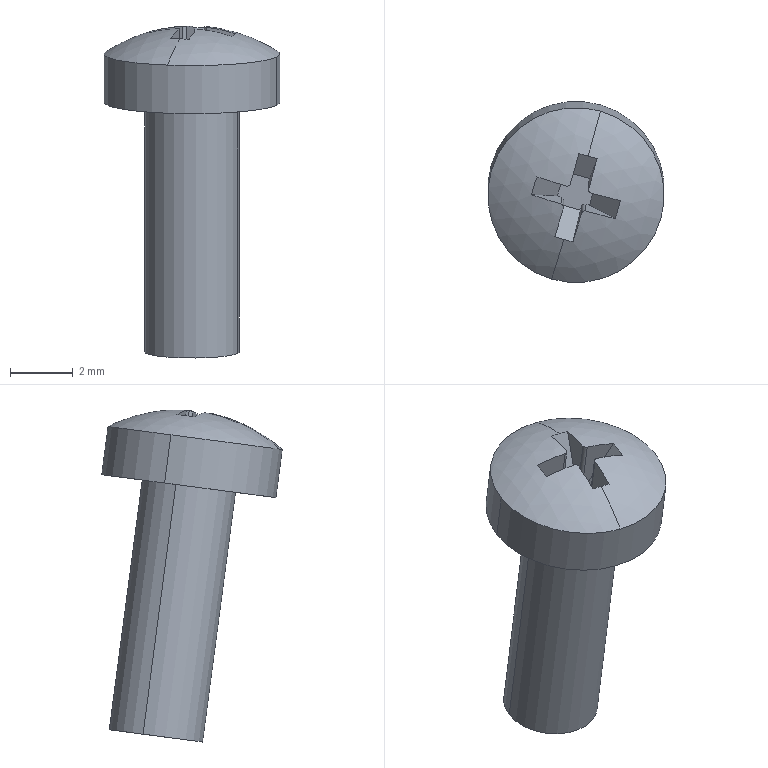Component | SolidWorks | SeedingAssemblyA-1_cross recessed pan head screws gb-12 | 1 solid | 25 faces | box 5.6 x 5.75 x 10.55 mm | volume 102 mm3 | plane 15 | cylinder 8 | sphere 2 | commonest cylinder face diameters 0.2 x4 5.6 x2 3 x2
STEP:
#1=COLOUR_RGB('',0.7922,0.8196,0.9333);
#2=FILL_AREA_STYLE_COLOUR('',#1);
#3=FILL_AREA_STYLE('',(#2));
#4=SURFACE_STYLE_FILL_AREA(#3);
#5=SURFACE_SIDE_STYLE('',(#4));
#6=SURFACE_STYLE_USAGE(.BOTH.,#5);
#7=PRESENTATION_STYLE_ASSIGNMENT((#6));
#8=CARTESIAN_POINT('',(3.542,-4.184,-2.825));
#9=VERTEX_POINT('',#8);
#10=CARTESIAN_POINT('',(3.466,-4.048,-2.807));
#11=VERTEX_POINT('',#10);
#12=CARTESIAN_POINT('',(3.572,-4.079,-2.811));
#13=DIRECTION('',(-0.,0.1306,-0.9914));
#14=DIRECTION('',(0.9609,-0.2744,-0.03615));
#15=AXIS2_PLACEMENT_3D('',#12,#13,#14);
#16=CIRCLE('',#15,0.1102);
#17=EDGE_CURVE('',#9,#11,#16,.T.);
#18=ORIENTED_EDGE('',*,*,#17,.T.);
#19=CARTESIAN_POINT('',(3.466,-4.04,-2.868));
#20=VERTEX_POINT('',#19);
#21=CARTESIAN_POINT('',(3.466,-4.029,-2.95));
#22=DIRECTION('',(-0.,0.1306,-0.9914));
#23=VECTOR('',#22,39.37);
#24=LINE('',#21,#23);
#25=EDGE_CURVE('',#11,#20,#24,.T.);
#26=ORIENTED_EDGE('',*,*,#25,.T.);
#27=CARTESIAN_POINT('',(3.678,-4.101,-2.876));
#28=VERTEX_POINT('',#27);
#29=CARTESIAN_POINT('',(3.572,-4.071,-2.872));
#30=DIRECTION('',(-0.,0.1306,-0.9914));
#31=DIRECTION('',(0.9609,-0.2744,-0.03615));
#32=AXIS2_PLACEMENT_3D('',#29,#30,#31);
#33=CIRCLE('',#32,0.1102);
#34=EDGE_CURVE('',#28,#20,#33,.T.);
#35=ORIENTED_EDGE('',*,*,#34,.F.);
#36=CARTESIAN_POINT('',(3.678,-4.109,-2.815));
#37=VERTEX_POINT('',#36);
#38=CARTESIAN_POINT('',(3.678,-4.09,-2.958));
#39=DIRECTION('',(-0.,0.1306,-0.9914));
#40=VECTOR('',#39,39.37);
#41=LINE('',#38,#40);
#42=EDGE_CURVE('',#37,#28,#41,.T.);
#43=ORIENTED_EDGE('',*,*,#42,.F.);
#44=CARTESIAN_POINT('',(3.572,-4.079,-2.811));
#45=DIRECTION('',(-0.,0.1306,-0.9914));
#46=DIRECTION('',(0.9609,-0.2744,-0.03615));
#47=AXIS2_PLACEMENT_3D('',#44,#45,#46);
#48=CIRCLE('',#47,0.1102);
#49=EDGE_CURVE('',#37,#9,#48,.T.);
#50=ORIENTED_EDGE('',*,*,#49,.T.);
#51=EDGE_LOOP('',(#18,#26,#35,#43,#50));
#52=FACE_OUTER_BOUND('',#51,.T.);
#53=CARTESIAN_POINT('',(3.572,-4.06,-2.954));
#54=DIRECTION('',(-0.,0.1306,-0.9914));
#55=DIRECTION('',(0.9609,-0.2744,-0.03615));
#56=AXIS2_PLACEMENT_3D('',#53,#54,#55);
#57=CYLINDRICAL_SURFACE('',#56,0.1102);
#58=ADVANCED_FACE('',(#52),#57,.T.);
#59=CARTESIAN_POINT('',(3.629,-4.087,-2.874));
#60=VERTEX_POINT('',#59);
#61=CARTESIAN_POINT('',(3.515,-4.054,-2.869));
#62=VERTEX_POINT('',#61);
#63=CARTESIAN_POINT('',(3.572,-4.071,-2.872));
#64=DIRECTION('',(-0.,0.1306,-0.9914));
#65=DIRECTION('',(0.9609,-0.2744,-0.03615));
#66=AXIS2_PLACEMENT_3D('',#63,#64,#65);
#67=CIRCLE('',#66,0.05906);
#68=EDGE_CURVE('',#60,#62,#67,.T.);
#69=ORIENTED_EDGE('',*,*,#68,.T.);
#70=CARTESIAN_POINT('',(3.515,-4.013,-3.182));
#71=VERTEX_POINT('',#70);
#72=CARTESIAN_POINT('',(3.515,-4.043,-2.952));
#73=DIRECTION('',(-0.,0.1306,-0.9914));
#74=VECTOR('',#73,39.37);
#75=LINE('',#72,#74);
#76=EDGE_CURVE('',#62,#71,#75,.T.);
#77=ORIENTED_EDGE('',*,*,#76,.T.);
#78=CARTESIAN_POINT('',(3.629,-4.046,-3.186));
#79=VERTEX_POINT('',#78);
#80=CARTESIAN_POINT('',(3.572,-4.029,-3.184));
#81=DIRECTION('',(-0.,0.1306,-0.9914));
#82=DIRECTION('',(0.9609,-0.2744,-0.03615));
#83=AXIS2_PLACEMENT_3D('',#80,#81,#82);
#84=CIRCLE('',#83,0.05906);
#85=EDGE_CURVE('',#79,#71,#84,.T.);
#86=ORIENTED_EDGE('',*,*,#85,.F.);
#87=CARTESIAN_POINT('',(3.629,-4.076,-2.956));
#88=DIRECTION('',(-0.,0.1306,-0.9914));
#89=VECTOR('',#88,39.37);
#90=LINE('',#87,#89);
#91=EDGE_CURVE('',#60,#79,#90,.T.);
#92=ORIENTED_EDGE('',*,*,#91,.F.);
#93=EDGE_LOOP('',(#69,#77,#86,#92));
#94=FACE_OUTER_BOUND('',#93,.T.);
#95=CARTESIAN_POINT('',(3.572,-4.06,-2.954));
#96=DIRECTION('',(-0.,0.1306,-0.9914));
#97=DIRECTION('',(0.9609,-0.2744,-0.03615));
#98=AXIS2_PLACEMENT_3D('',#95,#96,#97);
#99=CYLINDRICAL_SURFACE('',#98,0.05906);
#100=ADVANCED_FACE('',(#94),#99,.T.);
#101=CARTESIAN_POINT('',(3.576,-4.027,-2.779));
#102=VERTEX_POINT('',#101);
#103=CARTESIAN_POINT('',(3.587,-4.03,-2.779));
#104=VERTEX_POINT('',#103);
#105=CARTESIAN_POINT('',(3.561,-4.099,-2.955));
#106=DIRECTION('',(0.2397,0.8904,-0.387));
#107=DIRECTION('',(0.1384,0.3633,0.9214));
#108=AXIS2_PLACEMENT_3D('',#105,#106,#107);
#109=CIRCLE('',#108,0.1911);
#110=EDGE_CURVE('',#102,#104,#109,.T.);
#111=ORIENTED_EDGE('',*,*,#110,.T.);
#112=CARTESIAN_POINT('',(3.603,-3.973,-2.798));
#113=VERTEX_POINT('',#112);
#114=CARTESIAN_POINT('',(3.572,-4.057,-2.973));
#115=DIRECTION('',(-0.9609,0.2744,0.03615));
#116=DIRECTION('',(-0.2746,-0.9616,0.));
#117=AXIS2_PLACEMENT_3D('',#114,#115,#116);
#118=CIRCLE('',#117,0.1969);
#119=EDGE_CURVE('',#104,#113,#118,.T.);
#120=ORIENTED_EDGE('',*,*,#119,.T.);
#121=CARTESIAN_POINT('',(3.572,-4.079,-2.811));
#122=DIRECTION('',(-0.,0.1306,-0.9914));
#123=DIRECTION('',(0.9609,-0.2744,-0.03615));
#124=AXIS2_PLACEMENT_3D('',#121,#122,#123);
#125=CIRCLE('',#124,0.1102);
#126=EDGE_CURVE('',#11,#113,#125,.T.);
#127=ORIENTED_EDGE('',*,*,#126,.F.);
#128=ORIENTED_EDGE('',*,*,#17,.F.);
#129=CARTESIAN_POINT('',(3.557,-4.134,-2.792));
#130=VERTEX_POINT('',#129);
#131=CARTESIAN_POINT('',(3.572,-4.057,-2.973));
#132=DIRECTION('',(0.9609,-0.2744,-0.03615));
#133=DIRECTION('',(0.2746,0.9616,0.));
#134=AXIS2_PLACEMENT_3D('',#131,#132,#133);
#135=CIRCLE('',#134,0.1969);
#136=EDGE_CURVE('',#130,#9,#135,.T.);
#137=ORIENTED_EDGE('',*,*,#136,.F.);
#138=CARTESIAN_POINT('',(3.546,-4.13,-2.792));
#139=VERTEX_POINT('',#138);
#140=CARTESIAN_POINT('',(3.583,-4.021,-2.945));
#141=DIRECTION('',(-0.2397,-0.7598,-0.6044));
#142=DIRECTION('',(0.1384,0.5894,-0.7959));
#143=AXIS2_PLACEMENT_3D('',#140,#141,#142);
#144=CIRCLE('',#143,0.1911);
#145=EDGE_CURVE('',#130,#139,#144,.T.);
#146=ORIENTED_EDGE('',*,*,#145,.T.);
#147=CARTESIAN_POINT('',(3.556,-4.095,-2.78));
#148=VERTEX_POINT('',#147);
#149=CARTESIAN_POINT('',(3.561,-4.054,-2.973));
#150=DIRECTION('',(-0.9609,0.2744,0.03615));
#151=DIRECTION('',(-0.2768,-0.9527,-0.1255));
#152=AXIS2_PLACEMENT_3D('',#149,#150,#151);
#153=CIRCLE('',#152,0.1965);
#154=EDGE_CURVE('',#139,#148,#153,.T.);
#155=ORIENTED_EDGE('',*,*,#154,.T.);
#156=CARTESIAN_POINT('',(3.554,-4.09,-2.78));
#157=VERTEX_POINT('',#156);
#158=CARTESIAN_POINT('',(3.556,-4.095,-2.78));
#159=CARTESIAN_POINT('',(3.557,-4.094,-2.78));
#160=CARTESIAN_POINT('',(3.557,-4.094,-2.78));
#161=CARTESIAN_POINT('',(3.557,-4.093,-2.78));
#162=CARTESIAN_POINT('',(3.557,-4.093,-2.78));
#163=CARTESIAN_POINT('',(3.556,-4.092,-2.78));
#164=CARTESIAN_POINT('',(3.556,-4.092,-2.78));
#165=CARTESIAN_POINT('',(3.556,-4.092,-2.78));
#166=CARTESIAN_POINT('',(3.556,-4.091,-2.78));
#167=CARTESIAN_POINT('',(3.556,-4.091,-2.78));
#168=CARTESIAN_POINT('',(3.555,-4.091,-2.78));
#169=CARTESIAN_POINT('',(3.555,-4.09,-2.78));
#170=CARTESIAN_POINT('',(3.555,-4.09,-2.78));
#171=CARTESIAN_POINT('',(3.554,-4.09,-2.78));
#172=CARTESIAN_POINT('',(3.554,-4.09,-2.78));
#173=CARTESIAN_POINT('',(3.554,-4.09,-2.78));
#174=B_SPLINE_CURVE_WITH_KNOTS('',3,(#158,#159,#160,#161,#162,#163,#164,#165,#166,#167,#168,#169,#170,#171,#172,#173),.UNSPECIFIED.,.F.,.F.,(4,3,3,3,3,4),(0.,0.00003353,0.00006707,0.0001005,0.0001339,0.0001564),.UNSPECIFIED.);
#175=EDGE_CURVE('',#148,#157,#174,.T.);
#176=ORIENTED_EDGE('',*,*,#175,.T.);
#177=CARTESIAN_POINT('',(3.517,-4.078,-2.785));
#178=VERTEX_POINT('',#177);
#179=CARTESIAN_POINT('',(3.569,-4.068,-2.975));
#180=DIRECTION('',(-0.2768,-0.9527,-0.1255));
#181=DIRECTION('',(0.9609,-0.2744,-0.03615));
#182=AXIS2_PLACEMENT_3D('',#179,#180,#181);
#183=CIRCLE('',#182,0.1965);
#184=EDGE_CURVE('',#157,#178,#183,.T.);
#185=ORIENTED_EDGE('',*,*,#184,.T.);
#186=CARTESIAN_POINT('',(3.523,-4.056,-2.782));
#187=VERTEX_POINT('',#186);
#188=CARTESIAN_POINT('',(3.611,-4.072,-2.951));
#189=DIRECTION('',(-0.8322,0.303,-0.4644));
#190=DIRECTION('',(-0.4805,0.02413,0.8767));
#191=AXIS2_PLACEMENT_3D('',#188,#189,#190);
#192=CIRCLE('',#191,0.1911);
#193=EDGE_CURVE('',#178,#187,#192,.T.);
#194=ORIENTED_EDGE('',*,*,#193,.T.);
#195=CARTESIAN_POINT('',(3.56,-4.067,-2.777));
#196=VERTEX_POINT('',#195);
#197=CARTESIAN_POINT('',(3.575,-4.046,-2.972));
#198=DIRECTION('',(0.2768,0.9527,0.1255));
#199=DIRECTION('',(-0.9609,0.2744,0.03615));
#200=AXIS2_PLACEMENT_3D('',#197,#198,#199);
#201=CIRCLE('',#200,0.1965);
#202=EDGE_CURVE('',#187,#196,#201,.T.);
#203=ORIENTED_EDGE('',*,*,#202,.T.);
#204=CARTESIAN_POINT('',(3.565,-4.065,-2.777));
#205=VERTEX_POINT('',#204);
#206=CARTESIAN_POINT('',(3.56,-4.067,-2.777));
#207=CARTESIAN_POINT('',(3.561,-4.067,-2.777));
#208=CARTESIAN_POINT('',(3.561,-4.067,-2.777));
#209=CARTESIAN_POINT('',(3.562,-4.067,-2.777));
#210=CARTESIAN_POINT('',(3.562,-4.067,-2.777));
#211=CARTESIAN_POINT('',(3.562,-4.067,-2.777));
#212=CARTESIAN_POINT('',(3.563,-4.067,-2.777));
#213=CARTESIAN_POINT('',(3.563,-4.067,-2.777));
#214=CARTESIAN_POINT('',(3.564,-4.067,-2.777));
#215=CARTESIAN_POINT('',(3.564,-4.066,-2.777));
#216=CARTESIAN_POINT('',(3.564,-4.066,-2.777));
#217=CARTESIAN_POINT('',(3.565,-4.066,-2.777));
#218=CARTESIAN_POINT('',(3.565,-4.065,-2.777));
#219=CARTESIAN_POINT('',(3.565,-4.065,-2.777));
#220=CARTESIAN_POINT('',(3.565,-4.065,-2.777));
#221=CARTESIAN_POINT('',(3.565,-4.065,-2.777));
#222=B_SPLINE_CURVE_WITH_KNOTS('',3,(#206,#207,#208,#209,#210,#211,#212,#213,#214,#215,#216,#217,#218,#219,#220,#221),.UNSPECIFIED.,.F.,.F.,(4,3,3,3,3,4),(0.,0.00003353,0.00006707,0.0001005,0.0001339,0.0001564),.UNSPECIFIED.);
#223=EDGE_CURVE('',#196,#205,#222,.T.);
#224=ORIENTED_EDGE('',*,*,#223,.T.);
#225=CARTESIAN_POINT('',(3.561,-4.054,-2.973));
#226=DIRECTION('',(-0.9609,0.2744,0.03615));
#227=DIRECTION('',(-0.2768,-0.9527,-0.1255));
#228=AXIS2_PLACEMENT_3D('',#225,#226,#227);
#229=CIRCLE('',#228,0.1965);
#230=EDGE_CURVE('',#205,#102,#229,.T.);
#231=ORIENTED_EDGE('',*,*,#230,.T.);
#232=EDGE_LOOP('',(#111,#120,#127,#128,#137,#146,#155,#176,#185,#194,#203,#224,#231));
#233=FACE_OUTER_BOUND('',#232,.T.);
#234=CARTESIAN_POINT('',(3.572,-4.057,-2.973));
#235=DIRECTION('',(-0.9609,0.2744,0.03615));
#236=DIRECTION('',(-0.2768,-0.9527,-0.1255));
#237=AXIS2_PLACEMENT_3D('',#234,#235,#236);
#238=SPHERICAL_SURFACE('',#237,0.1969);
#239=ADVANCED_FACE('',(#233),#238,.T.);
#240=ORIENTED_EDGE('',*,*,#119,.F.);
#241=CARTESIAN_POINT('',(3.599,-4.033,-2.779));
#242=VERTEX_POINT('',#241);
#243=CARTESIAN_POINT('',(3.561,-4.099,-2.955));
#244=DIRECTION('',(0.2397,0.8904,-0.387));
#245=DIRECTION('',(0.1384,0.3633,0.9214));
#246=AXIS2_PLACEMENT_3D('',#243,#244,#245);
#247=CIRCLE('',#246,0.1911);
#248=EDGE_CURVE('',#104,#242,#247,.T.);
#249=ORIENTED_EDGE('',*,*,#248,.T.);
#250=CARTESIAN_POINT('',(3.588,-4.071,-2.777));
#251=VERTEX_POINT('',#250);
#252=CARTESIAN_POINT('',(3.583,-4.06,-2.974));
#253=DIRECTION('',(0.9609,-0.2744,-0.03615));
#254=DIRECTION('',(0.,0.1306,-0.9914));
#255=AXIS2_PLACEMENT_3D('',#252,#253,#254);
#256=CIRCLE('',#255,0.1965);
#257=EDGE_CURVE('',#242,#251,#256,.T.);
#258=ORIENTED_EDGE('',*,*,#257,.T.);
#259=CARTESIAN_POINT('',(3.591,-4.076,-2.778));
#260=VERTEX_POINT('',#259);
#261=CARTESIAN_POINT('',(3.588,-4.071,-2.777));
#262=CARTESIAN_POINT('',(3.588,-4.071,-2.777));
#263=CARTESIAN_POINT('',(3.588,-4.072,-2.777));
#264=CARTESIAN_POINT('',(3.588,-4.072,-2.777));
#265=CARTESIAN_POINT('',(3.588,-4.073,-2.777));
#266=CARTESIAN_POINT('',(3.588,-4.073,-2.778));
#267=CARTESIAN_POINT('',(3.588,-4.074,-2.778));
#268=CARTESIAN_POINT('',(3.588,-4.074,-2.778));
#269=CARTESIAN_POINT('',(3.588,-4.074,-2.778));
#270=CARTESIAN_POINT('',(3.589,-4.075,-2.778));
#271=CARTESIAN_POINT('',(3.589,-4.075,-2.778));
#272=CARTESIAN_POINT('',(3.589,-4.075,-2.778));
#273=CARTESIAN_POINT('',(3.59,-4.076,-2.778));
#274=CARTESIAN_POINT('',(3.59,-4.076,-2.778));
#275=CARTESIAN_POINT('',(3.59,-4.076,-2.778));
#276=CARTESIAN_POINT('',(3.591,-4.076,-2.778));
#277=B_SPLINE_CURVE_WITH_KNOTS('',3,(#261,#262,#263,#264,#265,#266,#267,#268,#269,#270,#271,#272,#273,#274,#275,#276),.UNSPECIFIED.,.F.,.F.,(4,3,3,3,3,4),(0.,0.00003353,0.00006707,0.0001005,0.0001339,0.0001564),.UNSPECIFIED.);
#278=EDGE_CURVE('',#251,#260,#277,.T.);
#279=ORIENTED_EDGE('',*,*,#278,.T.);
#280=CARTESIAN_POINT('',(3.628,-4.086,-2.786));
#281=VERTEX_POINT('',#280);
#282=CARTESIAN_POINT('',(3.575,-4.046,-2.972));
#283=DIRECTION('',(0.2768,0.9527,0.1255));
#284=DIRECTION('',(-0.9609,0.2744,0.03615));
#285=AXIS2_PLACEMENT_3D('',#282,#283,#284);
#286=CIRCLE('',#285,0.1965);
#287=EDGE_CURVE('',#260,#281,#286,.T.);
#288=ORIENTED_EDGE('',*,*,#287,.T.);
#289=CARTESIAN_POINT('',(3.621,-4.108,-2.789));
#290=VERTEX_POINT('',#289);
#291=CARTESIAN_POINT('',(3.533,-4.049,-2.948));
#292=DIRECTION('',(0.8322,-0.1724,-0.527));
#293=DIRECTION('',(-0.4805,0.2503,-0.8405));
#294=AXIS2_PLACEMENT_3D('',#291,#292,#293);
#295=CIRCLE('',#294,0.1911);
#296=EDGE_CURVE('',#281,#290,#295,.T.);
#297=ORIENTED_EDGE('',*,*,#296,.T.);
#298=CARTESIAN_POINT('',(3.584,-4.098,-2.781));
#299=VERTEX_POINT('',#298);
#300=CARTESIAN_POINT('',(3.569,-4.068,-2.975));
#301=DIRECTION('',(-0.2768,-0.9527,-0.1255));
#302=DIRECTION('',(0.9609,-0.2744,-0.03615));
#303=AXIS2_PLACEMENT_3D('',#300,#301,#302);
#304=CIRCLE('',#303,0.1965);
#305=EDGE_CURVE('',#290,#299,#304,.T.);
#306=ORIENTED_EDGE('',*,*,#305,.T.);
#307=CARTESIAN_POINT('',(3.579,-4.101,-2.781));
#308=VERTEX_POINT('',#307);
#309=CARTESIAN_POINT('',(3.584,-4.098,-2.781));
#310=CARTESIAN_POINT('',(3.584,-4.098,-2.781));
#311=CARTESIAN_POINT('',(3.583,-4.098,-2.781));
#312=CARTESIAN_POINT('',(3.583,-4.098,-2.781));
#313=CARTESIAN_POINT('',(3.582,-4.098,-2.781));
#314=CARTESIAN_POINT('',(3.582,-4.098,-2.781));
#315=CARTESIAN_POINT('',(3.581,-4.099,-2.781));
#316=CARTESIAN_POINT('',(3.581,-4.099,-2.781));
#317=CARTESIAN_POINT('',(3.581,-4.099,-2.781));
#318=CARTESIAN_POINT('',(3.58,-4.099,-2.781));
#319=CARTESIAN_POINT('',(3.58,-4.1,-2.781));
#320=CARTESIAN_POINT('',(3.58,-4.1,-2.781));
#321=CARTESIAN_POINT('',(3.579,-4.1,-2.781));
#322=CARTESIAN_POINT('',(3.579,-4.1,-2.781));
#323=CARTESIAN_POINT('',(3.579,-4.101,-2.781));
#324=CARTESIAN_POINT('',(3.579,-4.101,-2.781));
#325=B_SPLINE_CURVE_WITH_KNOTS('',3,(#309,#310,#311,#312,#313,#314,#315,#316,#317,#318,#319,#320,#321,#322,#323,#324),.UNSPECIFIED.,.F.,.F.,(4,3,3,3,3,4),(0.,0.00003353,0.00006707,0.0001005,0.0001339,0.0001564),.UNSPECIFIED.);
#326=EDGE_CURVE('',#299,#308,#325,.T.);
#327=ORIENTED_EDGE('',*,*,#326,.T.);
#328=CARTESIAN_POINT('',(3.568,-4.137,-2.793));
#329=VERTEX_POINT('',#328);
#330=CARTESIAN_POINT('',(3.583,-4.06,-2.974));
#331=DIRECTION('',(0.9609,-0.2744,-0.03615));
#332=DIRECTION('',(0.,0.1306,-0.9914));
#333=AXIS2_PLACEMENT_3D('',#330,#331,#332);
#334=CIRCLE('',#333,0.1965);
#335=EDGE_CURVE('',#308,#329,#334,.T.);
#336=ORIENTED_EDGE('',*,*,#335,.T.);
#337=CARTESIAN_POINT('',(3.583,-4.021,-2.945));
#338=DIRECTION('',(-0.2397,-0.7598,-0.6044));
#339=DIRECTION('',(0.1384,0.5894,-0.7959));
#340=AXIS2_PLACEMENT_3D('',#337,#338,#339);
#341=CIRCLE('',#340,0.1911);
#342=EDGE_CURVE('',#329,#130,#341,.T.);
#343=ORIENTED_EDGE('',*,*,#342,.T.);
#344=ORIENTED_EDGE('',*,*,#136,.T.);
#345=ORIENTED_EDGE('',*,*,#49,.F.);
#346=CARTESIAN_POINT('',(3.572,-4.079,-2.811));
#347=DIRECTION('',(-0.,0.1306,-0.9914));
#348=DIRECTION('',(0.9609,-0.2744,-0.03615));
#349=AXIS2_PLACEMENT_3D('',#346,#347,#348);
#350=CIRCLE('',#349,0.1102);
#351=EDGE_CURVE('',#113,#37,#350,.T.);
#352=ORIENTED_EDGE('',*,*,#351,.F.);
#353=EDGE_LOOP('',(#240,#249,#258,#279,#288,#297,#306,#327,#336,#343,#344,#345,#352));
#354=FACE_OUTER_BOUND('',#353,.T.);
#355=CARTESIAN_POINT('',(3.572,-4.057,-2.973));
#356=DIRECTION('',(-0.9609,0.2744,0.03615));
#357=DIRECTION('',(-0.2768,-0.9527,-0.1255));
#358=AXIS2_PLACEMENT_3D('',#355,#356,#357);
#359=SPHERICAL_SURFACE('',#358,0.1969);
#360=ADVANCED_FACE('',(#354),#359,.T.);
#361=ORIENTED_EDGE('',*,*,#85,.T.);
#362=CARTESIAN_POINT('',(3.572,-4.029,-3.184));
#363=DIRECTION('',(-0.,0.1306,-0.9914));
#364=DIRECTION('',(0.9609,-0.2744,-0.03615));
#365=AXIS2_PLACEMENT_3D('',#362,#363,#364);
#366=CIRCLE('',#365,0.05906);
#367=EDGE_CURVE('',#71,#79,#366,.T.);
#368=ORIENTED_EDGE('',*,*,#367,.T.);
#369=EDGE_LOOP('',(#361,#368));
#370=FACE_OUTER_BOUND('',#369,.T.);
#371=CARTESIAN_POINT('',(3.556,-4.086,-3.191));
#372=DIRECTION('',(-0.,0.1306,-0.9914));
#373=DIRECTION('',(0.9609,-0.2744,-0.03615));
#374=AXIS2_PLACEMENT_3D('',#371,#372,#373);
#375=PLANE('',#374);
#376=ADVANCED_FACE('',(#370),#375,.T.);
#377=ORIENTED_EDGE('',*,*,#76,.F.);
#378=CARTESIAN_POINT('',(3.572,-4.071,-2.872));
#379=DIRECTION('',(-0.,0.1306,-0.9914));
#380=DIRECTION('',(0.9609,-0.2744,-0.03615));
#381=AXIS2_PLACEMENT_3D('',#378,#379,#380);
#382=CIRCLE('',#381,0.05906);
#383=EDGE_CURVE('',#62,#60,#382,.T.);
#384=ORIENTED_EDGE('',*,*,#383,.T.);
#385=ORIENTED_EDGE('',*,*,#91,.T.);
#386=ORIENTED_EDGE('',*,*,#367,.F.);
#387=EDGE_LOOP('',(#377,#384,#385,#386));
#388=FACE_OUTER_BOUND('',#387,.T.);
#389=CARTESIAN_POINT('',(3.572,-4.06,-2.954));
#390=DIRECTION('',(-0.,0.1306,-0.9914));
#391=DIRECTION('',(0.9609,-0.2744,-0.03615));
#392=AXIS2_PLACEMENT_3D('',#389,#390,#391);
#393=CYLINDRICAL_SURFACE('',#392,0.05906);
#394=ADVANCED_FACE('',(#388),#393,.T.);
#395=ORIENTED_EDGE('',*,*,#34,.T.);
#396=CARTESIAN_POINT('',(3.572,-4.071,-2.872));
#397=DIRECTION('',(-0.,0.1306,-0.9914));
#398=DIRECTION('',(0.9609,-0.2744,-0.03615));
#399=AXIS2_PLACEMENT_3D('',#396,#397,#398);
#400=CIRCLE('',#399,0.1102);
#401=EDGE_CURVE('',#20,#28,#400,.T.);
#402=ORIENTED_EDGE('',*,*,#401,.T.);
#403=EDGE_LOOP('',(#395,#402));
#404=FACE_OUTER_BOUND('',#403,.T.);
#405=ORIENTED_EDGE('',*,*,#68,.F.);
#406=ORIENTED_EDGE('',*,*,#383,.F.);
#407=EDGE_LOOP('',(#405,#406));
#408=FACE_BOUND('',#407,.T.);
#409=CARTESIAN_POINT('',(3.552,-4.138,-2.88));
#410=DIRECTION('',(-0.,0.1306,-0.9914));
#411=DIRECTION('',(0.9609,-0.2744,-0.03615));
#412=AXIS2_PLACEMENT_3D('',#409,#410,#411);
#413=PLANE('',#412);
#414=ADVANCED_FACE('',(#404,#408),#413,.T.);
#415=ORIENTED_EDGE('',*,*,#25,.F.);
#416=ORIENTED_EDGE('',*,*,#126,.T.);
#417=ORIENTED_EDGE('',*,*,#351,.T.);
#418=ORIENTED_EDGE('',*,*,#42,.T.);
#419=ORIENTED_EDGE('',*,*,#401,.F.);
#420=EDGE_LOOP('',(#415,#416,#417,#418,#419));
#421=FACE_OUTER_BOUND('',#420,.T.);
#422=CARTESIAN_POINT('',(3.572,-4.06,-2.954));
#423=DIRECTION('',(-0.,0.1306,-0.9914));
#424=DIRECTION('',(0.9609,-0.2744,-0.03615));
#425=AXIS2_PLACEMENT_3D('',#422,#423,#424);
#426=CYLINDRICAL_SURFACE('',#425,0.1102);
#427=ADVANCED_FACE('',(#421),#426,.T.);
#428=ORIENTED_EDGE('',*,*,#184,.F.);
#429=CARTESIAN_POINT('',(3.554,-4.081,-2.844));
#430=VERTEX_POINT('',#429);
#431=CARTESIAN_POINT('',(3.554,-4.081,-2.844));
#432=DIRECTION('',(-0.,0.1306,-0.9914));
#433=VECTOR('',#432,39.37);
#434=LINE('',#431,#433);
#435=EDGE_CURVE('',#157,#430,#434,.T.);
#436=ORIENTED_EDGE('',*,*,#435,.T.);
#437=CARTESIAN_POINT('',(3.549,-4.08,-2.844));
#438=VERTEX_POINT('',#437);
#439=CARTESIAN_POINT('',(3.557,-4.082,-2.845));
#440=DIRECTION('',(-0.9609,0.2744,0.03615));
#441=VECTOR('',#440,39.37);
#442=LINE('',#439,#441);
#443=EDGE_CURVE('',#430,#438,#442,.T.);
#444=ORIENTED_EDGE('',*,*,#443,.T.);
#445=CARTESIAN_POINT('',(3.512,-4.078,-2.777));
#446=DIRECTION('',(-0.4805,0.02413,0.8767));
#447=VECTOR('',#446,39.37);
#448=LINE('',#445,#447);
#449=EDGE_CURVE('',#438,#178,#448,.T.);
#450=ORIENTED_EDGE('',*,*,#449,.T.);
#451=EDGE_LOOP('',(#428,#436,#444,#450));
#452=FACE_OUTER_BOUND('',#451,.T.);
#453=CARTESIAN_POINT('',(3.557,-4.082,-2.845));
#454=DIRECTION('',(0.2768,0.9527,0.1255));
#455=DIRECTION('',(0.9609,-0.2744,-0.03615));
#456=AXIS2_PLACEMENT_3D('',#453,#454,#455);
#457=PLANE('',#456);
#458=ADVANCED_FACE('',(#452),#457,.T.);
#459=ORIENTED_EDGE('',*,*,#449,.F.);
#460=CARTESIAN_POINT('',(3.555,-4.057,-2.841));
#461=VERTEX_POINT('',#460);
#462=CARTESIAN_POINT('',(3.549,-4.08,-2.844));
#463=DIRECTION('',(0.2768,0.9527,0.1255));
#464=VECTOR('',#463,39.37);
#465=LINE('',#462,#464);
#466=EDGE_CURVE('',#438,#461,#465,.T.);
#467=ORIENTED_EDGE('',*,*,#466,.T.);
#468=CARTESIAN_POINT('',(3.557,-4.057,-2.845));
#469=DIRECTION('',(-0.4805,0.02413,0.8767));
#470=VECTOR('',#469,39.37);
#471=LINE('',#468,#470);
#472=EDGE_CURVE('',#461,#187,#471,.T.);
#473=ORIENTED_EDGE('',*,*,#472,.T.);
#474=ORIENTED_EDGE('',*,*,#193,.F.);
#475=EDGE_LOOP('',(#459,#467,#473,#474));
#476=FACE_OUTER_BOUND('',#475,.T.);
#477=CARTESIAN_POINT('',(3.515,-4.067,-2.776));
#478=DIRECTION('',(0.8322,-0.303,0.4644));
#479=DIRECTION('',(-0.4805,0.02413,0.8767));
#480=AXIS2_PLACEMENT_3D('',#477,#478,#479);
#481=PLANE('',#480);
#482=ADVANCED_FACE('',(#476),#481,.T.);
#483=CARTESIAN_POINT('',(3.56,-4.059,-2.841));
#484=VERTEX_POINT('',#483);
#485=CARTESIAN_POINT('',(3.564,-4.06,-2.842));
#486=DIRECTION('',(0.9609,-0.2744,-0.03615));
#487=VECTOR('',#486,39.37);
#488=LINE('',#485,#487);
#489=EDGE_CURVE('',#461,#484,#488,.T.);
#490=ORIENTED_EDGE('',*,*,#489,.T.);
#491=CARTESIAN_POINT('',(3.56,-4.059,-2.841));
#492=DIRECTION('',(0.,-0.1306,0.9914));
#493=VECTOR('',#492,39.37);
#494=LINE('',#491,#493);
#495=EDGE_CURVE('',#484,#196,#494,.T.);
#496=ORIENTED_EDGE('',*,*,#495,.T.);
#497=ORIENTED_EDGE('',*,*,#202,.F.);
#498=ORIENTED_EDGE('',*,*,#472,.F.);
#499=EDGE_LOOP('',(#490,#496,#497,#498));
#500=FACE_OUTER_BOUND('',#499,.T.);
#501=CARTESIAN_POINT('',(3.564,-4.06,-2.842));
#502=DIRECTION('',(-0.2768,-0.9527,-0.1255));
#503=DIRECTION('',(-0.9609,0.2744,0.03615));
#504=AXIS2_PLACEMENT_3D('',#501,#502,#503);
#505=PLANE('',#504);
#506=ADVANCED_FACE('',(#500),#505,.T.);
#507=ORIENTED_EDGE('',*,*,#230,.F.);
#508=CARTESIAN_POINT('',(3.565,-4.056,-2.841));
#509=VERTEX_POINT('',#508);
#510=CARTESIAN_POINT('',(3.565,-4.056,-2.841));
#511=DIRECTION('',(-0.,0.1306,-0.9914));
#512=VECTOR('',#511,39.37);
#513=LINE('',#510,#512);
#514=EDGE_CURVE('',#205,#509,#513,.T.);
#515=ORIENTED_EDGE('',*,*,#514,.T.);
#516=CARTESIAN_POINT('',(3.567,-4.051,-2.84));
#517=VERTEX_POINT('',#516);
#518=CARTESIAN_POINT('',(3.564,-4.06,-2.842));
#519=DIRECTION('',(0.2768,0.9527,0.1255));
#520=VECTOR('',#519,39.37);
#521=LINE('',#518,#520);
#522=EDGE_CURVE('',#509,#517,#521,.T.);
#523=ORIENTED_EDGE('',*,*,#522,.T.);
#524=CARTESIAN_POINT('',(3.577,-4.023,-2.77));
#525=DIRECTION('',(0.1384,0.3633,0.9214));
#526=VECTOR('',#525,39.37);
#527=LINE('',#524,#526);
#528=EDGE_CURVE('',#517,#102,#527,.T.);
#529=ORIENTED_EDGE('',*,*,#528,.T.);
#530=EDGE_LOOP('',(#507,#515,#523,#529));
#531=FACE_OUTER_BOUND('',#530,.T.);
#532=CARTESIAN_POINT('',(3.564,-4.06,-2.842));
#533=DIRECTION('',(0.9609,-0.2744,-0.03615));
#534=DIRECTION('',(-0.2768,-0.9527,-0.1255));
#535=AXIS2_PLACEMENT_3D('',#532,#533,#534);
#536=PLANE('',#535);
#537=ADVANCED_FACE('',(#531),#536,.T.);
#538=ORIENTED_EDGE('',*,*,#528,.F.);
#539=CARTESIAN_POINT('',(3.589,-4.058,-2.841));
#540=VERTEX_POINT('',#539);
#541=CARTESIAN_POINT('',(3.567,-4.051,-2.84));
#542=DIRECTION('',(0.9609,-0.2744,-0.03615));
#543=VECTOR('',#542,39.37);
#544=LINE('',#541,#543);
#545=EDGE_CURVE('',#517,#540,#544,.T.);
#546=ORIENTED_EDGE('',*,*,#545,.T.);
#547=CARTESIAN_POINT('',(3.589,-4.059,-2.845));
#548=DIRECTION('',(0.1384,0.3633,0.9214));
#549=VECTOR('',#548,39.37);
#550=LINE('',#547,#549);
#551=EDGE_CURVE('',#540,#242,#550,.T.);
#552=ORIENTED_EDGE('',*,*,#551,.T.);
#553=ORIENTED_EDGE('',*,*,#248,.F.);
#554=ORIENTED_EDGE('',*,*,#110,.F.);
#555=EDGE_LOOP('',(#538,#546,#552,#553,#554));
#556=FACE_OUTER_BOUND('',#555,.T.);
#557=CARTESIAN_POINT('',(3.588,-4.027,-2.771));
#558=DIRECTION('',(-0.2397,-0.8904,0.387));
#559=DIRECTION('',(0.1384,0.3633,0.9214));
#560=AXIS2_PLACEMENT_3D('',#557,#558,#559);
#561=PLANE('',#560);
#562=ADVANCED_FACE('',(#556),#561,.T.);
#563=CARTESIAN_POINT('',(3.588,-4.063,-2.842));
#564=VERTEX_POINT('',#563);
#565=CARTESIAN_POINT('',(3.587,-4.066,-2.842));
#566=DIRECTION('',(-0.2768,-0.9527,-0.1255));
#567=VECTOR('',#566,39.37);
#568=LINE('',#565,#567);
#569=EDGE_CURVE('',#540,#564,#568,.T.);
#570=ORIENTED_EDGE('',*,*,#569,.T.);
#571=CARTESIAN_POINT('',(3.588,-4.063,-2.842));
#572=DIRECTION('',(0.,-0.1306,0.9914));
#573=VECTOR('',#572,39.37);
#574=LINE('',#571,#573);
#575=EDGE_CURVE('',#564,#251,#574,.T.);
#576=ORIENTED_EDGE('',*,*,#575,.T.);
#577=ORIENTED_EDGE('',*,*,#257,.F.);
#578=ORIENTED_EDGE('',*,*,#551,.F.);
#579=EDGE_LOOP('',(#570,#576,#577,#578));
#580=FACE_OUTER_BOUND('',#579,.T.);
#581=CARTESIAN_POINT('',(3.587,-4.066,-2.842));
#582=DIRECTION('',(-0.9609,0.2744,0.03615));
#583=DIRECTION('',(-0.,0.1306,-0.9914));
#584=AXIS2_PLACEMENT_3D('',#581,#582,#583);
#585=PLANE('',#584);
#586=ADVANCED_FACE('',(#580),#585,.T.);
#587=ORIENTED_EDGE('',*,*,#287,.F.);
#588=CARTESIAN_POINT('',(3.591,-4.067,-2.843));
#589=VERTEX_POINT('',#588);
#590=CARTESIAN_POINT('',(3.591,-4.067,-2.843));
#591=DIRECTION('',(-0.,0.1306,-0.9914));
#592=VECTOR('',#591,39.37);
#593=LINE('',#590,#592);
#594=EDGE_CURVE('',#260,#589,#593,.T.);
#595=ORIENTED_EDGE('',*,*,#594,.T.);
#596=CARTESIAN_POINT('',(3.595,-4.069,-2.843));
#597=VERTEX_POINT('',#596);
#598=CARTESIAN_POINT('',(3.587,-4.066,-2.842));
#599=DIRECTION('',(0.9609,-0.2744,-0.03615));
#600=VECTOR('',#599,39.37);
#601=LINE('',#598,#600);
#602=EDGE_CURVE('',#589,#597,#601,.T.);
#603=ORIENTED_EDGE('',*,*,#602,.T.);
#604=CARTESIAN_POINT('',(3.632,-4.088,-2.779));
#605=DIRECTION('',(0.4805,-0.2503,0.8405));
#606=VECTOR('',#605,39.37);
#607=LINE('',#604,#606);
#608=EDGE_CURVE('',#597,#281,#607,.T.);
#609=ORIENTED_EDGE('',*,*,#608,.T.);
#610=EDGE_LOOP('',(#587,#595,#603,#609));
#611=FACE_OUTER_BOUND('',#610,.T.);
#612=CARTESIAN_POINT('',(3.587,-4.066,-2.842));
#613=DIRECTION('',(-0.2768,-0.9527,-0.1255));
#614=DIRECTION('',(-0.9609,0.2744,0.03615));
#615=AXIS2_PLACEMENT_3D('',#612,#613,#614);
#616=PLANE('',#615);
#617=ADVANCED_FACE('',(#611),#616,.T.);
#618=ORIENTED_EDGE('',*,*,#608,.F.);
#619=CARTESIAN_POINT('',(3.589,-4.091,-2.846));
#620=VERTEX_POINT('',#619);
#621=CARTESIAN_POINT('',(3.589,-4.091,-2.846));
#622=DIRECTION('',(-0.2768,-0.9527,-0.1255));
#623=VECTOR('',#622,39.37);
#624=LINE('',#621,#623);
#625=EDGE_CURVE('',#597,#620,#624,.T.);
#626=ORIENTED_EDGE('',*,*,#625,.T.);
#627=CARTESIAN_POINT('',(3.587,-4.09,-2.85));
#628=DIRECTION('',(0.4805,-0.2503,0.8405));
#629=VECTOR('',#628,39.37);
#630=LINE('',#627,#629);
#631=EDGE_CURVE('',#620,#290,#630,.T.);
#632=ORIENTED_EDGE('',*,*,#631,.T.);
#633=ORIENTED_EDGE('',*,*,#296,.F.);
#634=EDGE_LOOP('',(#618,#626,#632,#633));
#635=FACE_OUTER_BOUND('',#634,.T.);
#636=CARTESIAN_POINT('',(3.629,-4.099,-2.78));
#637=DIRECTION('',(-0.8322,0.1724,0.527));
#638=DIRECTION('',(-0.4805,0.2503,-0.8405));
#639=AXIS2_PLACEMENT_3D('',#636,#637,#638);
#640=PLANE('',#639);
#641=ADVANCED_FACE('',(#635),#640,.T.);
#642=CARTESIAN_POINT('',(3.584,-4.09,-2.846));
#643=VERTEX_POINT('',#642);
#644=CARTESIAN_POINT('',(3.58,-4.089,-2.845));
#645=DIRECTION('',(-0.9609,0.2744,0.03615));
#646=VECTOR('',#645,39.37);
#647=LINE('',#644,#646);
#648=EDGE_CURVE('',#620,#643,#647,.T.);
#649=ORIENTED_EDGE('',*,*,#648,.T.);
#650=CARTESIAN_POINT('',(3.584,-4.09,-2.846));
#651=DIRECTION('',(0.,-0.1306,0.9914));
#652=VECTOR('',#651,39.37);
#653=LINE('',#650,#652);
#654=EDGE_CURVE('',#643,#299,#653,.T.);
#655=ORIENTED_EDGE('',*,*,#654,.T.);
#656=ORIENTED_EDGE('',*,*,#305,.F.);
#657=ORIENTED_EDGE('',*,*,#631,.F.);
#658=EDGE_LOOP('',(#649,#655,#656,#657));
#659=FACE_OUTER_BOUND('',#658,.T.);
#660=CARTESIAN_POINT('',(3.58,-4.089,-2.845));
#661=DIRECTION('',(0.2768,0.9527,0.1255));
#662=DIRECTION('',(0.9609,-0.2744,-0.03615));
#663=AXIS2_PLACEMENT_3D('',#660,#661,#662);
#664=PLANE('',#663);
#665=ADVANCED_FACE('',(#659),#664,.T.);
#666=ORIENTED_EDGE('',*,*,#335,.F.);
#667=CARTESIAN_POINT('',(3.579,-4.093,-2.846));
#668=VERTEX_POINT('',#667);
#669=CARTESIAN_POINT('',(3.579,-4.093,-2.846));
#670=DIRECTION('',(-0.,0.1306,-0.9914));
#671=VECTOR('',#670,39.37);
#672=LINE('',#669,#671);
#673=EDGE_CURVE('',#308,#668,#672,.T.);
#674=ORIENTED_EDGE('',*,*,#673,.T.);
#675=CARTESIAN_POINT('',(3.578,-4.097,-2.847));
#676=VERTEX_POINT('',#675);
#677=CARTESIAN_POINT('',(3.58,-4.089,-2.845));
#678=DIRECTION('',(-0.2768,-0.9527,-0.1255));
#679=VECTOR('',#678,39.37);
#680=LINE('',#677,#679);
#681=EDGE_CURVE('',#668,#676,#680,.T.);
#682=ORIENTED_EDGE('',*,*,#681,.T.);
#683=CARTESIAN_POINT('',(3.567,-4.142,-2.786));
#684=DIRECTION('',(-0.1384,-0.5894,0.7959));
#685=VECTOR('',#684,39.37);
#686=LINE('',#683,#685);
#687=EDGE_CURVE('',#676,#329,#686,.T.);
#688=ORIENTED_EDGE('',*,*,#687,.T.);
#689=EDGE_LOOP('',(#666,#674,#682,#688));
#690=FACE_OUTER_BOUND('',#689,.T.);
#691=CARTESIAN_POINT('',(3.58,-4.089,-2.845));
#692=DIRECTION('',(-0.9609,0.2744,0.03615));
#693=DIRECTION('',(-0.,0.1306,-0.9914));
#694=AXIS2_PLACEMENT_3D('',#691,#692,#693);
#695=PLANE('',#694);
#696=ADVANCED_FACE('',(#690),#695,.T.);
#697=ORIENTED_EDGE('',*,*,#687,.F.);
#698=CARTESIAN_POINT('',(3.555,-4.091,-2.846));
#699=VERTEX_POINT('',#698);
#700=CARTESIAN_POINT('',(3.555,-4.091,-2.846));
#701=DIRECTION('',(-0.9609,0.2744,0.03615));
#702=VECTOR('',#701,39.37);
#703=LINE('',#700,#702);
#704=EDGE_CURVE('',#676,#699,#703,.T.);
#705=ORIENTED_EDGE('',*,*,#704,.T.);
#706=CARTESIAN_POINT('',(3.556,-4.088,-2.849));
#707=DIRECTION('',(-0.1384,-0.5894,0.7959));
#708=VECTOR('',#707,39.37);
#709=LINE('',#706,#708);
#710=EDGE_CURVE('',#699,#139,#709,.T.);
#711=ORIENTED_EDGE('',*,*,#710,.T.);
#712=ORIENTED_EDGE('',*,*,#145,.F.);
#713=ORIENTED_EDGE('',*,*,#342,.F.);
#714=EDGE_LOOP('',(#697,#705,#711,#712,#713));
#715=FACE_OUTER_BOUND('',#714,.T.);
#716=CARTESIAN_POINT('',(3.556,-4.139,-2.785));
#717=DIRECTION('',(0.2397,0.7598,0.6044));
#718=DIRECTION('',(0.1384,0.5894,-0.7959));
#719=AXIS2_PLACEMENT_3D('',#716,#717,#718);
#720=PLANE('',#719);
#721=ADVANCED_FACE('',(#715),#720,.T.);
#722=CARTESIAN_POINT('',(3.556,-4.086,-2.845));
#723=VERTEX_POINT('',#722);
#724=CARTESIAN_POINT('',(3.557,-4.082,-2.845));
#725=DIRECTION('',(0.2768,0.9527,0.1255));
#726=VECTOR('',#725,39.37);
#727=LINE('',#724,#726);
#728=EDGE_CURVE('',#699,#723,#727,.T.);
#729=ORIENTED_EDGE('',*,*,#728,.T.);
#730=CARTESIAN_POINT('',(3.556,-4.086,-2.845));
#731=DIRECTION('',(0.,-0.1306,0.9914));
#732=VECTOR('',#731,39.37);
#733=LINE('',#730,#732);
#734=EDGE_CURVE('',#723,#148,#733,.T.);
#735=ORIENTED_EDGE('',*,*,#734,.T.);
#736=ORIENTED_EDGE('',*,*,#154,.F.);
#737=ORIENTED_EDGE('',*,*,#710,.F.);
#738=EDGE_LOOP('',(#729,#735,#736,#737));
#739=FACE_OUTER_BOUND('',#738,.T.);
#740=CARTESIAN_POINT('',(3.557,-4.082,-2.845));
#741=DIRECTION('',(0.9609,-0.2744,-0.03615));
#742=DIRECTION('',(-0.2768,-0.9527,-0.1255));
#743=AXIS2_PLACEMENT_3D('',#740,#741,#742);
#744=PLANE('',#743);
#745=ADVANCED_FACE('',(#739),#744,.T.);
#746=ORIENTED_EDGE('',*,*,#443,.F.);
#747=CARTESIAN_POINT('',(3.553,-4.085,-2.845));
#748=DIRECTION('',(-0.,0.1306,-0.9914));
#749=DIRECTION('',(-0.9609,0.2744,0.03615));
#750=AXIS2_PLACEMENT_3D('',#747,#748,#749);
#751=CIRCLE('',#750,0.003937);
#752=EDGE_CURVE('',#430,#723,#751,.T.);
#753=ORIENTED_EDGE('',*,*,#752,.T.);
#754=ORIENTED_EDGE('',*,*,#728,.F.);
#755=ORIENTED_EDGE('',*,*,#704,.F.);
#756=ORIENTED_EDGE('',*,*,#681,.F.);
#757=CARTESIAN_POINT('',(3.583,-4.094,-2.846));
#758=DIRECTION('',(-0.,0.1306,-0.9914));
#759=DIRECTION('',(-0.9609,0.2744,0.03615));
#760=AXIS2_PLACEMENT_3D('',#757,#758,#759);
#761=CIRCLE('',#760,0.003937);
#762=EDGE_CURVE('',#668,#643,#761,.T.);
#763=ORIENTED_EDGE('',*,*,#762,.T.);
#764=ORIENTED_EDGE('',*,*,#648,.F.);
#765=ORIENTED_EDGE('',*,*,#625,.F.);
#766=ORIENTED_EDGE('',*,*,#602,.F.);
#767=CARTESIAN_POINT('',(3.592,-4.064,-2.842));
#768=DIRECTION('',(-0.,0.1306,-0.9914));
#769=DIRECTION('',(-0.9609,0.2744,0.03615));
#770=AXIS2_PLACEMENT_3D('',#767,#768,#769);
#771=CIRCLE('',#770,0.003937);
#772=EDGE_CURVE('',#589,#564,#771,.T.);
#773=ORIENTED_EDGE('',*,*,#772,.T.);
#774=ORIENTED_EDGE('',*,*,#569,.F.);
#775=ORIENTED_EDGE('',*,*,#545,.F.);
#776=ORIENTED_EDGE('',*,*,#522,.F.);
#777=CARTESIAN_POINT('',(3.561,-4.055,-2.841));
#778=DIRECTION('',(-0.,0.1306,-0.9914));
#779=DIRECTION('',(-0.9609,0.2744,0.03615));
#780=AXIS2_PLACEMENT_3D('',#777,#778,#779);
#781=CIRCLE('',#780,0.003937);
#782=EDGE_CURVE('',#509,#484,#781,.T.);
#783=ORIENTED_EDGE('',*,*,#782,.T.);
#784=ORIENTED_EDGE('',*,*,#489,.F.);
#785=ORIENTED_EDGE('',*,*,#466,.F.);
#786=EDGE_LOOP('',(#746,#753,#754,#755,#756,#763,#764,#765,#766,#773,#774,#775,#776,#783,#784,#785));
#787=FACE_OUTER_BOUND('',#786,.T.);
#788=CARTESIAN_POINT('',(3.557,-4.082,-2.845));
#789=DIRECTION('',(0.,-0.1306,0.9914));
#790=DIRECTION('',(-0.9609,0.2744,0.03615));
#791=AXIS2_PLACEMENT_3D('',#788,#789,#790);
#792=PLANE('',#791);
#793=ADVANCED_FACE('',(#787),#792,.T.);
#794=ORIENTED_EDGE('',*,*,#782,.F.);
#795=ORIENTED_EDGE('',*,*,#514,.F.);
#796=ORIENTED_EDGE('',*,*,#223,.F.);
#797=ORIENTED_EDGE('',*,*,#495,.F.);
#798=EDGE_LOOP('',(#794,#795,#796,#797));
#799=FACE_OUTER_BOUND('',#798,.T.);
#800=CARTESIAN_POINT('',(3.561,-4.055,-2.841));
#801=DIRECTION('',(0.,-0.1306,0.9914));
#802=DIRECTION('',(-0.9609,0.2744,0.03615));
#803=AXIS2_PLACEMENT_3D('',#800,#801,#802);
#804=CYLINDRICAL_SURFACE('',#803,0.003937);
#805=ADVANCED_FACE('',(#799),#804,.T.);
#806=ORIENTED_EDGE('',*,*,#772,.F.);
#807=ORIENTED_EDGE('',*,*,#594,.F.);
#808=ORIENTED_EDGE('',*,*,#278,.F.);
#809=ORIENTED_EDGE('',*,*,#575,.F.);
#810=EDGE_LOOP('',(#806,#807,#808,#809));
#811=FACE_OUTER_BOUND('',#810,.T.);
#812=CARTESIAN_POINT('',(3.592,-4.064,-2.842));
#813=DIRECTION('',(0.,-0.1306,0.9914));
#814=DIRECTION('',(-0.9609,0.2744,0.03615));
#815=AXIS2_PLACEMENT_3D('',#812,#813,#814);
#816=CYLINDRICAL_SURFACE('',#815,0.003937);
#817=ADVANCED_FACE('',(#811),#816,.T.);
#818=ORIENTED_EDGE('',*,*,#752,.F.);
#819=ORIENTED_EDGE('',*,*,#435,.F.);
#820=ORIENTED_EDGE('',*,*,#175,.F.);
#821=ORIENTED_EDGE('',*,*,#734,.F.);
#822=EDGE_LOOP('',(#818,#819,#820,#821));
#823=FACE_OUTER_BOUND('',#822,.T.);
#824=CARTESIAN_POINT('',(3.553,-4.085,-2.845));
#825=DIRECTION('',(0.,-0.1306,0.9914));
#826=DIRECTION('',(-0.9609,0.2744,0.03615));
#827=AXIS2_PLACEMENT_3D('',#824,#825,#826);
#828=CYLINDRICAL_SURFACE('',#827,0.003937);
#829=ADVANCED_FACE('',(#823),#828,.T.);
#830=ORIENTED_EDGE('',*,*,#762,.F.);
#831=ORIENTED_EDGE('',*,*,#673,.F.);
#832=ORIENTED_EDGE('',*,*,#326,.F.);
#833=ORIENTED_EDGE('',*,*,#654,.F.);
#834=EDGE_LOOP('',(#830,#831,#832,#833));
#835=FACE_OUTER_BOUND('',#834,.T.);
#836=CARTESIAN_POINT('',(3.583,-4.094,-2.846));
#837=DIRECTION('',(0.,-0.1306,0.9914));
#838=DIRECTION('',(-0.9609,0.2744,0.03615));
#839=AXIS2_PLACEMENT_3D('',#836,#837,#838);
#840=CYLINDRICAL_SURFACE('',#839,0.003937);
#841=ADVANCED_FACE('',(#835),#840,.T.);
#842=CLOSED_SHELL('',(#58,#100,#239,#360,#376,#394,#414,#427,#458,#482,#506,#537,#562,#586,#617,#641,#665,#696,#721,#745,#793,#805,#817,#829,#841));
#843=MANIFOLD_SOLID_BREP('',#842);
#844=STYLED_ITEM('',(#7),#843);
#845=(LENGTH_UNIT()NAMED_UNIT(*)SI_UNIT($,.METRE.));
#846=LENGTH_MEASURE_WITH_UNIT(LENGTH_MEASURE(0.0254),#845);
#847=DIMENSIONAL_EXPONENTS(1.,0.,0.,0.,0.,0.,0.);
#848=(CONVERSION_BASED_UNIT('',#846)LENGTH_UNIT()NAMED_UNIT(#847));
#849=UNCERTAINTY_MEASURE_WITH_UNIT(LENGTH_MEASURE(0.00001),#848,'','');
#850=(NAMED_UNIT(*)PLANE_ANGLE_UNIT()SI_UNIT($,.RADIAN.));
#851=(NAMED_UNIT(*)SI_UNIT($,.STERADIAN.)SOLID_ANGLE_UNIT());
#852=(GEOMETRIC_REPRESENTATION_CONTEXT(3)GLOBAL_UNCERTAINTY_ASSIGNED_CONTEXT((#849))GLOBAL_UNIT_ASSIGNED_CONTEXT((#848,#850,#851))REPRESENTATION_CONTEXT('',''));
#853=MECHANICAL_DESIGN_GEOMETRIC_PRESENTATION_REPRESENTATION('',(#844),#852);
#854=PRESENTATION_LAYER_ASSIGNMENT('','',(#844));
#855=CARTESIAN_POINT('',(0.,0.,0.));
#856=DIRECTION('',(0.,0.,1.));
#857=DIRECTION('',(1.,0.,0.));
#858=AXIS2_PLACEMENT_3D('',#855,#856,#857);
#859=(LENGTH_UNIT()NAMED_UNIT(*)SI_UNIT($,.METRE.));
#860=LENGTH_MEASURE_WITH_UNIT(LENGTH_MEASURE(0.0254),#859);
#861=DIMENSIONAL_EXPONENTS(1.,0.,0.,0.,0.,0.,0.);
#862=(CONVERSION_BASED_UNIT('',#860)LENGTH_UNIT()NAMED_UNIT(#861));
#863=UNCERTAINTY_MEASURE_WITH_UNIT(LENGTH_MEASURE(0.00001),#862,'','');
#864=(NAMED_UNIT(*)PLANE_ANGLE_UNIT()SI_UNIT($,.RADIAN.));
#865=(NAMED_UNIT(*)SI_UNIT($,.STERADIAN.)SOLID_ANGLE_UNIT());
#866=(GEOMETRIC_REPRESENTATION_CONTEXT(3)GLOBAL_UNCERTAINTY_ASSIGNED_CONTEXT((#863))GLOBAL_UNIT_ASSIGNED_CONTEXT((#862,#864,#865))REPRESENTATION_CONTEXT('',''));
#867=ADVANCED_BREP_SHAPE_REPRESENTATION('',(#843,#858),#866);